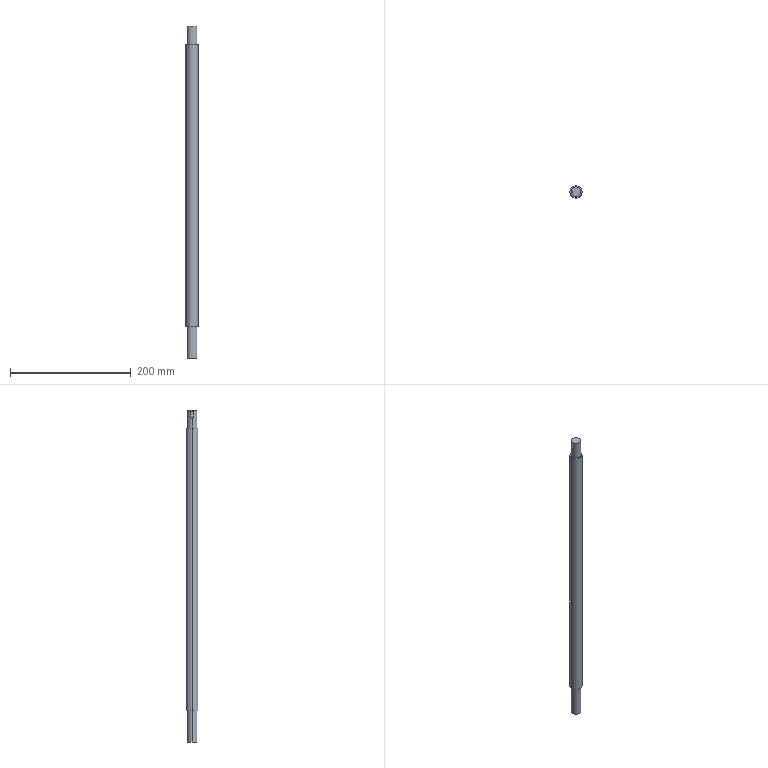Component | SolidWorks | LeadScrew-1 | 1 solid | 16 faces | box 20 x 20 x 550.64 mm | volume 163626 mm3 | cylinder 9 | plane 7 | commonest cylinder face diameters 16 x4 4 x3 20 x2
build123d program:
from build123d import *

# Parameters (mm, degrees)
SKETCH1_R           = 10
BOSS_EXTRUDE1_DEPTH = 529
SKETCH2_R           = 10
SKETCH2_R_2         = 8
CUT_EXTRUDE1_DEPTH  = 30
CUT_EXTRUDE2_START  = -30
SKETCH3_R           = 10
SKETCH3_R_2         = 8
CUT_EXTRUDE2_DEPTH  = 30
MOVE_FACE1_BY       = 21.644
CUT_EXTRUDE3_DEPTH  = 3


with BuildPart() as part:
    # Sketch1 → Boss-Extrude1 (new body)
    with BuildSketch(Plane.XY):
        with Locations((0, -208.707)):
            Circle(SKETCH1_R)
    extrude(amount=BOSS_EXTRUDE1_DEPTH)

    # Sketch2 → Cut-Extrude1 (cut)
    with BuildSketch(Plane(origin=(0, 0, 0), x_dir=(-1, 0, 0), z_dir=(0, 0, -1))):
        with Locations((0, -208.707)):
            Circle(SKETCH2_R)
        with Locations((0, -208.707)):
            Circle(SKETCH2_R_2, mode=Mode.SUBTRACT)
    extrude(amount=-CUT_EXTRUDE1_DEPTH, mode=Mode.SUBTRACT)

    # Sketch3 → Cut-Extrude2 (cut)
    with BuildSketch(Plane.XY.offset(529).offset(CUT_EXTRUDE2_START)):
        with Locations(Location((0, -208.707, 0), (0, 0, 180))):
            Circle(SKETCH3_R)
        with Locations(Location((0, -208.707, 0), (0, 0, 180))):
            Circle(SKETCH3_R_2, mode=Mode.SUBTRACT)
    extrude(amount=CUT_EXTRUDE2_DEPTH, mode=Mode.SUBTRACT)

    # Move Face1: a face moved outward by 21.644
    extrude(part.faces().sort_by_distance((0, -208.707, 529))[0], amount=MOVE_FACE1_BY, dir=(0, 0, 1))

    # Sketch4 → Cut-Extrude3 (cut)
    with BuildSketch(Plane(origin=(8, 0, 0), x_dir=(0, 0, -1), z_dir=(1, 0, 0))):
        with BuildLine():
            Line((-12, -206.707), (-4, -206.707))
            ThreePointArc((-4, -206.707), (-2, -208.707), (-4, -210.707))
            Line((-4, -210.707), (-12, -210.707))
            ThreePointArc((-12, -210.707), (-14, -208.707), (-12, -206.707))
        make_face()
    extrude(amount=-CUT_EXTRUDE3_DEPTH, mode=Mode.SUBTRACT)


solid = part.part

# Placed as in the assembly
solid = solid.moved(Location((0, 0, -102), (-180, 0, 180)))
STEP:
#1=CARTESIAN_POINT('',(-0.1969,-8.217,-4.094));
#2=VERTEX_POINT('',#1);
#3=CARTESIAN_POINT('',(-0.1969,-8.138,-4.173));
#4=VERTEX_POINT('',#3);
#5=CARTESIAN_POINT('',(-0.1969,-8.217,-4.173));
#6=DIRECTION('',(-1.,0.,0.));
#7=DIRECTION('',(0.,0.,1.));
#8=AXIS2_PLACEMENT_3D('',#5,#6,#7);
#9=CIRCLE('',#8,0.07874);
#10=EDGE_CURVE('',#2,#4,#9,.T.);
#11=ORIENTED_EDGE('',*,*,#10,.F.);
#12=CARTESIAN_POINT('',(-0.315,-8.217,-4.094));
#13=VERTEX_POINT('',#12);
#14=CARTESIAN_POINT('',(-0.1969,-8.217,-4.094));
#15=DIRECTION('',(-1.,0.,0.));
#16=VECTOR('',#15,39.37);
#17=LINE('',#14,#16);
#18=EDGE_CURVE('',#2,#13,#17,.T.);
#19=ORIENTED_EDGE('',*,*,#18,.T.);
#20=CARTESIAN_POINT('',(-0.305,-8.138,-4.173));
#21=VERTEX_POINT('',#20);
#22=CARTESIAN_POINT('',(-0.315,-8.217,-4.094));
#23=CARTESIAN_POINT('',(-0.315,-8.212,-4.094));
#24=CARTESIAN_POINT('',(-0.3148,-8.206,-4.095));
#25=CARTESIAN_POINT('',(-0.3143,-8.196,-4.097));
#26=CARTESIAN_POINT('',(-0.314,-8.191,-4.099));
#27=CARTESIAN_POINT('',(-0.3126,-8.177,-4.104));
#28=CARTESIAN_POINT('',(-0.3113,-8.168,-4.11));
#29=CARTESIAN_POINT('',(-0.3093,-8.158,-4.121));
#30=CARTESIAN_POINT('',(-0.3087,-8.154,-4.125));
#31=CARTESIAN_POINT('',(-0.3075,-8.149,-4.134));
#32=CARTESIAN_POINT('',(-0.3069,-8.146,-4.138));
#33=CARTESIAN_POINT('',(-0.306,-8.142,-4.148));
#34=CARTESIAN_POINT('',(-0.3056,-8.141,-4.153));
#35=CARTESIAN_POINT('',(-0.3051,-8.139,-4.163));
#36=CARTESIAN_POINT('',(-0.305,-8.138,-4.168));
#37=CARTESIAN_POINT('',(-0.305,-8.138,-4.173));
#38=B_SPLINE_CURVE_WITH_KNOTS('',3,(#22,#23,#24,#25,#26,#27,#28,#29,#30,#31,#32,#33,#34,#35,#36,#37),.UNSPECIFIED.,.F.,.F.,(4,2,2,2,2,2,2,4),(0.00314,0.003532,0.003924,0.004708,0.0051,0.005492,0.005884,0.006276),.UNSPECIFIED.);
#39=EDGE_CURVE('',#13,#21,#38,.T.);
#40=ORIENTED_EDGE('',*,*,#39,.T.);
#41=CARTESIAN_POINT('',(-0.1969,-8.138,-4.173));
#42=DIRECTION('',(-1.,0.,0.));
#43=VECTOR('',#42,39.37);
#44=LINE('',#41,#43);
#45=EDGE_CURVE('',#4,#21,#44,.T.);
#46=ORIENTED_EDGE('',*,*,#45,.F.);
#47=EDGE_LOOP('',(#11,#19,#40,#46));
#48=FACE_OUTER_BOUND('',#47,.T.);
#49=CARTESIAN_POINT('',(-0.1969,-8.217,-4.173));
#50=DIRECTION('',(-1.,0.,0.));
#51=DIRECTION('',(0.,0.,1.));
#52=AXIS2_PLACEMENT_3D('',#49,#50,#51);
#53=CYLINDRICAL_SURFACE('',#52,0.07874);
#54=ADVANCED_FACE('',(#48),#53,.F.);
#55=CARTESIAN_POINT('',(-0.315,-8.217,-23.661));
#56=VERTEX_POINT('',#55);
#57=CARTESIAN_POINT('',(0.315,-8.217,-23.661));
#58=VERTEX_POINT('',#57);
#59=CARTESIAN_POINT('',(0.,-8.217,-23.661));
#60=DIRECTION('',(0.,0.,-1.));
#61=DIRECTION('',(-1.,0.,0.));
#62=AXIS2_PLACEMENT_3D('',#59,#60,#61);
#63=CIRCLE('',#62,0.315);
#64=EDGE_CURVE('',#56,#58,#63,.T.);
#65=ORIENTED_EDGE('',*,*,#64,.T.);
#66=CARTESIAN_POINT('',(0.315,-8.217,-25.695));
#67=VERTEX_POINT('',#66);
#68=CARTESIAN_POINT('',(0.315,-8.217,-23.661));
#69=DIRECTION('',(0.,0.,-1.));
#70=VECTOR('',#69,39.37);
#71=LINE('',#68,#70);
#72=EDGE_CURVE('',#58,#67,#71,.T.);
#73=ORIENTED_EDGE('',*,*,#72,.T.);
#74=CARTESIAN_POINT('',(-0.315,-8.217,-25.695));
#75=VERTEX_POINT('',#74);
#76=CARTESIAN_POINT('',(0.,-8.217,-25.695));
#77=DIRECTION('',(0.,0.,-1.));
#78=DIRECTION('',(-1.,0.,0.));
#79=AXIS2_PLACEMENT_3D('',#76,#77,#78);
#80=CIRCLE('',#79,0.315);
#81=EDGE_CURVE('',#75,#67,#80,.T.);
#82=ORIENTED_EDGE('',*,*,#81,.F.);
#83=CARTESIAN_POINT('',(-0.315,-8.217,-23.661));
#84=DIRECTION('',(0.,0.,-1.));
#85=VECTOR('',#84,39.37);
#86=LINE('',#83,#85);
#87=EDGE_CURVE('',#56,#75,#86,.T.);
#88=ORIENTED_EDGE('',*,*,#87,.F.);
#89=EDGE_LOOP('',(#65,#73,#82,#88));
#90=FACE_OUTER_BOUND('',#89,.T.);
#91=CARTESIAN_POINT('',(0.,-8.217,-23.661));
#92=DIRECTION('',(0.,0.,-1.));
#93=DIRECTION('',(-1.,0.,0.));
#94=AXIS2_PLACEMENT_3D('',#91,#92,#93);
#95=CYLINDRICAL_SURFACE('',#94,0.315);
#96=ADVANCED_FACE('',(#90),#95,.T.);
#97=CARTESIAN_POINT('',(0.315,-8.217,-5.197));
#98=VERTEX_POINT('',#97);
#99=CARTESIAN_POINT('',(-0.315,-8.217,-5.197));
#100=VERTEX_POINT('',#99);
#101=CARTESIAN_POINT('',(0.,-8.217,-5.197));
#102=DIRECTION('',(0.,0.,1.));
#103=DIRECTION('',(1.,0.,0.));
#104=AXIS2_PLACEMENT_3D('',#101,#102,#103);
#105=CIRCLE('',#104,0.315);
#106=EDGE_CURVE('',#98,#100,#105,.T.);
#107=ORIENTED_EDGE('',*,*,#106,.T.);
#108=CARTESIAN_POINT('',(-0.315,-8.217,-4.567));
#109=VERTEX_POINT('',#108);
#110=CARTESIAN_POINT('',(-0.315,-8.217,-5.197));
#111=DIRECTION('',(0.,0.,1.));
#112=VECTOR('',#111,39.37);
#113=LINE('',#110,#112);
#114=EDGE_CURVE('',#100,#109,#113,.T.);
#115=ORIENTED_EDGE('',*,*,#114,.T.);
#116=CARTESIAN_POINT('',(-0.305,-8.138,-4.488));
#117=VERTEX_POINT('',#116);
#118=CARTESIAN_POINT('',(-0.305,-8.138,-4.488));
#119=CARTESIAN_POINT('',(-0.305,-8.138,-4.493));
#120=CARTESIAN_POINT('',(-0.3051,-8.139,-4.499));
#121=CARTESIAN_POINT('',(-0.3056,-8.141,-4.509));
#122=CARTESIAN_POINT('',(-0.306,-8.142,-4.514));
#123=CARTESIAN_POINT('',(-0.3069,-8.146,-4.523));
#124=CARTESIAN_POINT('',(-0.3075,-8.149,-4.528));
#125=CARTESIAN_POINT('',(-0.3087,-8.154,-4.536));
#126=CARTESIAN_POINT('',(-0.3094,-8.158,-4.54));
#127=CARTESIAN_POINT('',(-0.3113,-8.168,-4.551));
#128=CARTESIAN_POINT('',(-0.3126,-8.177,-4.557));
#129=CARTESIAN_POINT('',(-0.314,-8.191,-4.563));
#130=CARTESIAN_POINT('',(-0.3143,-8.196,-4.564));
#131=CARTESIAN_POINT('',(-0.3148,-8.207,-4.566));
#132=CARTESIAN_POINT('',(-0.315,-8.212,-4.567));
#133=CARTESIAN_POINT('',(-0.315,-8.217,-4.567));
#134=B_SPLINE_CURVE_WITH_KNOTS('',3,(#118,#119,#120,#121,#122,#123,#124,#125,#126,#127,#128,#129,#130,#131,#132,#133),.UNSPECIFIED.,.F.,.F.,(4,2,2,2,2,2,2,4),(0.,0.0003925,0.0007849,0.001177,0.00157,0.002355,0.002747,0.00314),.UNSPECIFIED.);
#135=EDGE_CURVE('',#117,#109,#134,.T.);
#136=ORIENTED_EDGE('',*,*,#135,.F.);
#137=CARTESIAN_POINT('',(-0.305,-8.138,-5.197));
#138=DIRECTION('',(0.,0.,-1.));
#139=VECTOR('',#138,39.37);
#140=LINE('',#137,#139);
#141=EDGE_CURVE('',#21,#117,#140,.T.);
#142=ORIENTED_EDGE('',*,*,#141,.F.);
#143=ORIENTED_EDGE('',*,*,#39,.F.);
#144=CARTESIAN_POINT('',(-0.315,-8.217,-4.016));
#145=VERTEX_POINT('',#144);
#146=CARTESIAN_POINT('',(-0.315,-8.217,-5.197));
#147=DIRECTION('',(0.,0.,1.));
#148=VECTOR('',#147,39.37);
#149=LINE('',#146,#148);
#150=EDGE_CURVE('',#13,#145,#149,.T.);
#151=ORIENTED_EDGE('',*,*,#150,.T.);
#152=CARTESIAN_POINT('',(0.315,-8.217,-4.016));
#153=VERTEX_POINT('',#152);
#154=CARTESIAN_POINT('',(0.,-8.217,-4.016));
#155=DIRECTION('',(0.,0.,1.));
#156=DIRECTION('',(1.,0.,0.));
#157=AXIS2_PLACEMENT_3D('',#154,#155,#156);
#158=CIRCLE('',#157,0.315);
#159=EDGE_CURVE('',#153,#145,#158,.T.);
#160=ORIENTED_EDGE('',*,*,#159,.F.);
#161=CARTESIAN_POINT('',(0.315,-8.217,-5.197));
#162=DIRECTION('',(0.,0.,1.));
#163=VECTOR('',#162,39.37);
#164=LINE('',#161,#163);
#165=EDGE_CURVE('',#98,#153,#164,.T.);
#166=ORIENTED_EDGE('',*,*,#165,.F.);
#167=EDGE_LOOP('',(#107,#115,#136,#142,#143,#151,#160,#166));
#168=FACE_OUTER_BOUND('',#167,.T.);
#169=CARTESIAN_POINT('',(0.,-8.217,-5.197));
#170=DIRECTION('',(0.,0.,1.));
#171=DIRECTION('',(1.,0.,0.));
#172=AXIS2_PLACEMENT_3D('',#169,#170,#171);
#173=CYLINDRICAL_SURFACE('',#172,0.315);
#174=ADVANCED_FACE('',(#168),#173,.T.);
#175=CARTESIAN_POINT('',(-0.3937,-8.217,-23.661));
#176=VERTEX_POINT('',#175);
#177=CARTESIAN_POINT('',(0.3937,-8.217,-23.661));
#178=VERTEX_POINT('',#177);
#179=CARTESIAN_POINT('',(0.,-8.217,-23.661));
#180=DIRECTION('',(0.,0.,-1.));
#181=DIRECTION('',(-1.,0.,0.));
#182=AXIS2_PLACEMENT_3D('',#179,#180,#181);
#183=CIRCLE('',#182,0.3937);
#184=EDGE_CURVE('',#176,#178,#183,.T.);
#185=ORIENTED_EDGE('',*,*,#184,.F.);
#186=CARTESIAN_POINT('',(-0.3937,-8.217,-5.197));
#187=VERTEX_POINT('',#186);
#188=CARTESIAN_POINT('',(-0.3937,-8.217,-24.843));
#189=DIRECTION('',(0.,0.,1.));
#190=VECTOR('',#189,39.37);
#191=LINE('',#188,#190);
#192=EDGE_CURVE('',#176,#187,#191,.T.);
#193=ORIENTED_EDGE('',*,*,#192,.T.);
#194=CARTESIAN_POINT('',(0.3937,-8.217,-5.197));
#195=VERTEX_POINT('',#194);
#196=CARTESIAN_POINT('',(0.,-8.217,-5.197));
#197=DIRECTION('',(0.,0.,1.));
#198=DIRECTION('',(1.,0.,0.));
#199=AXIS2_PLACEMENT_3D('',#196,#197,#198);
#200=CIRCLE('',#199,0.3937);
#201=EDGE_CURVE('',#195,#187,#200,.T.);
#202=ORIENTED_EDGE('',*,*,#201,.F.);
#203=CARTESIAN_POINT('',(0.3937,-8.217,-24.843));
#204=DIRECTION('',(0.,0.,1.));
#205=VECTOR('',#204,39.37);
#206=LINE('',#203,#205);
#207=EDGE_CURVE('',#178,#195,#206,.T.);
#208=ORIENTED_EDGE('',*,*,#207,.F.);
#209=EDGE_LOOP('',(#185,#193,#202,#208));
#210=FACE_OUTER_BOUND('',#209,.T.);
#211=CARTESIAN_POINT('',(0.,-8.217,-24.843));
#212=DIRECTION('',(0.,0.,1.));
#213=DIRECTION('',(1.,0.,0.));
#214=AXIS2_PLACEMENT_3D('',#211,#212,#213);
#215=CYLINDRICAL_SURFACE('',#214,0.3937);
#216=ADVANCED_FACE('',(#210),#215,.T.);
#217=ORIENTED_EDGE('',*,*,#192,.F.);
#218=CARTESIAN_POINT('',(0.,-8.217,-23.661));
#219=DIRECTION('',(0.,0.,-1.));
#220=DIRECTION('',(-1.,0.,0.));
#221=AXIS2_PLACEMENT_3D('',#218,#219,#220);
#222=CIRCLE('',#221,0.3937);
#223=EDGE_CURVE('',#178,#176,#222,.T.);
#224=ORIENTED_EDGE('',*,*,#223,.F.);
#225=ORIENTED_EDGE('',*,*,#207,.T.);
#226=CARTESIAN_POINT('',(0.,-8.217,-5.197));
#227=DIRECTION('',(0.,0.,1.));
#228=DIRECTION('',(1.,0.,0.));
#229=AXIS2_PLACEMENT_3D('',#226,#227,#228);
#230=CIRCLE('',#229,0.3937);
#231=EDGE_CURVE('',#187,#195,#230,.T.);
#232=ORIENTED_EDGE('',*,*,#231,.F.);
#233=EDGE_LOOP('',(#217,#224,#225,#232));
#234=FACE_OUTER_BOUND('',#233,.T.);
#235=CARTESIAN_POINT('',(0.,-8.217,-24.843));
#236=DIRECTION('',(0.,0.,1.));
#237=DIRECTION('',(1.,0.,0.));
#238=AXIS2_PLACEMENT_3D('',#235,#236,#237);
#239=CYLINDRICAL_SURFACE('',#238,0.3937);
#240=ADVANCED_FACE('',(#234),#239,.T.);
#241=ORIENTED_EDGE('',*,*,#106,.F.);
#242=CARTESIAN_POINT('',(0.,-8.217,-5.197));
#243=DIRECTION('',(0.,0.,1.));
#244=DIRECTION('',(1.,0.,0.));
#245=AXIS2_PLACEMENT_3D('',#242,#243,#244);
#246=CIRCLE('',#245,0.315);
#247=EDGE_CURVE('',#100,#98,#246,.T.);
#248=ORIENTED_EDGE('',*,*,#247,.F.);
#249=EDGE_LOOP('',(#241,#248));
#250=FACE_BOUND('',#249,.T.);
#251=ORIENTED_EDGE('',*,*,#201,.T.);
#252=ORIENTED_EDGE('',*,*,#231,.T.);
#253=EDGE_LOOP('',(#251,#252));
#254=FACE_OUTER_BOUND('',#253,.T.);
#255=CARTESIAN_POINT('',(0.,-8.217,-5.197));
#256=DIRECTION('',(0.,0.,1.));
#257=DIRECTION('',(1.,0.,0.));
#258=AXIS2_PLACEMENT_3D('',#255,#256,#257);
#259=PLANE('',#258);
#260=ADVANCED_FACE('',(#250,#254),#259,.T.);
#261=ORIENTED_EDGE('',*,*,#114,.F.);
#262=ORIENTED_EDGE('',*,*,#247,.T.);
#263=ORIENTED_EDGE('',*,*,#165,.T.);
#264=CARTESIAN_POINT('',(0.,-8.217,-4.016));
#265=DIRECTION('',(0.,0.,1.));
#266=DIRECTION('',(1.,0.,0.));
#267=AXIS2_PLACEMENT_3D('',#264,#265,#266);
#268=CIRCLE('',#267,0.315);
#269=EDGE_CURVE('',#145,#153,#268,.T.);
#270=ORIENTED_EDGE('',*,*,#269,.F.);
#271=ORIENTED_EDGE('',*,*,#150,.F.);
#272=CARTESIAN_POINT('',(-0.305,-8.296,-4.173));
#273=VERTEX_POINT('',#272);
#274=CARTESIAN_POINT('',(-0.305,-8.296,-4.173));
#275=CARTESIAN_POINT('',(-0.305,-8.296,-4.168));
#276=CARTESIAN_POINT('',(-0.3051,-8.295,-4.163));
#277=CARTESIAN_POINT('',(-0.3056,-8.293,-4.153));
#278=CARTESIAN_POINT('',(-0.306,-8.292,-4.148));
#279=CARTESIAN_POINT('',(-0.3069,-8.288,-4.138));
#280=CARTESIAN_POINT('',(-0.3075,-8.285,-4.134));
#281=CARTESIAN_POINT('',(-0.3087,-8.279,-4.125));
#282=CARTESIAN_POINT('',(-0.3094,-8.276,-4.121));
#283=CARTESIAN_POINT('',(-0.3113,-8.265,-4.11));
#284=CARTESIAN_POINT('',(-0.3126,-8.256,-4.104));
#285=CARTESIAN_POINT('',(-0.314,-8.242,-4.099));
#286=CARTESIAN_POINT('',(-0.3143,-8.237,-4.097));
#287=CARTESIAN_POINT('',(-0.3148,-8.227,-4.095));
#288=CARTESIAN_POINT('',(-0.315,-8.222,-4.094));
#289=CARTESIAN_POINT('',(-0.315,-8.217,-4.094));
#290=B_SPLINE_CURVE_WITH_KNOTS('',3,(#274,#275,#276,#277,#278,#279,#280,#281,#282,#283,#284,#285,#286,#287,#288,#289),.UNSPECIFIED.,.F.,.F.,(4,2,2,2,2,2,2,4),(0.,0.0003925,0.0007849,0.001177,0.00157,0.002355,0.002747,0.00314),.UNSPECIFIED.);
#291=EDGE_CURVE('',#273,#13,#290,.T.);
#292=ORIENTED_EDGE('',*,*,#291,.F.);
#293=CARTESIAN_POINT('',(-0.305,-8.296,-4.488));
#294=VERTEX_POINT('',#293);
#295=CARTESIAN_POINT('',(-0.305,-8.296,-5.197));
#296=DIRECTION('',(0.,0.,1.));
#297=VECTOR('',#296,39.37);
#298=LINE('',#295,#297);
#299=EDGE_CURVE('',#294,#273,#298,.T.);
#300=ORIENTED_EDGE('',*,*,#299,.F.);
#301=CARTESIAN_POINT('',(-0.315,-8.217,-4.567));
#302=CARTESIAN_POINT('',(-0.315,-8.222,-4.567));
#303=CARTESIAN_POINT('',(-0.3148,-8.227,-4.566));
#304=CARTESIAN_POINT('',(-0.3143,-8.237,-4.564));
#305=CARTESIAN_POINT('',(-0.314,-8.242,-4.563));
#306=CARTESIAN_POINT('',(-0.3126,-8.257,-4.557));
#307=CARTESIAN_POINT('',(-0.3113,-8.265,-4.551));
#308=CARTESIAN_POINT('',(-0.3093,-8.276,-4.54));
#309=CARTESIAN_POINT('',(-0.3087,-8.279,-4.536));
#310=CARTESIAN_POINT('',(-0.3075,-8.285,-4.528));
#311=CARTESIAN_POINT('',(-0.3069,-8.288,-4.523));
#312=CARTESIAN_POINT('',(-0.306,-8.292,-4.514));
#313=CARTESIAN_POINT('',(-0.3056,-8.293,-4.509));
#314=CARTESIAN_POINT('',(-0.3051,-8.295,-4.499));
#315=CARTESIAN_POINT('',(-0.305,-8.296,-4.493));
#316=CARTESIAN_POINT('',(-0.305,-8.296,-4.488));
#317=B_SPLINE_CURVE_WITH_KNOTS('',3,(#301,#302,#303,#304,#305,#306,#307,#308,#309,#310,#311,#312,#313,#314,#315,#316),.UNSPECIFIED.,.F.,.F.,(4,2,2,2,2,2,2,4),(0.00314,0.003532,0.003924,0.004708,0.0051,0.005492,0.005884,0.006276),.UNSPECIFIED.);
#318=EDGE_CURVE('',#109,#294,#317,.T.);
#319=ORIENTED_EDGE('',*,*,#318,.F.);
#320=EDGE_LOOP('',(#261,#262,#263,#270,#271,#292,#300,#319));
#321=FACE_OUTER_BOUND('',#320,.T.);
#322=CARTESIAN_POINT('',(0.,-8.217,-5.197));
#323=DIRECTION('',(0.,0.,1.));
#324=DIRECTION('',(1.,0.,0.));
#325=AXIS2_PLACEMENT_3D('',#322,#323,#324);
#326=CYLINDRICAL_SURFACE('',#325,0.315);
#327=ADVANCED_FACE('',(#321),#326,.T.);
#328=ORIENTED_EDGE('',*,*,#159,.T.);
#329=ORIENTED_EDGE('',*,*,#269,.T.);
#330=EDGE_LOOP('',(#328,#329));
#331=FACE_OUTER_BOUND('',#330,.T.);
#332=CARTESIAN_POINT('',(0.,-8.217,-4.016));
#333=DIRECTION('',(0.,0.,-1.));
#334=DIRECTION('',(-1.,0.,0.));
#335=AXIS2_PLACEMENT_3D('',#332,#333,#334);
#336=PLANE('',#335);
#337=ADVANCED_FACE('',(#331),#336,.F.);
#338=ORIENTED_EDGE('',*,*,#72,.F.);
#339=CARTESIAN_POINT('',(0.,-8.217,-23.661));
#340=DIRECTION('',(0.,0.,-1.));
#341=DIRECTION('',(-1.,0.,0.));
#342=AXIS2_PLACEMENT_3D('',#339,#340,#341);
#343=CIRCLE('',#342,0.315);
#344=EDGE_CURVE('',#58,#56,#343,.T.);
#345=ORIENTED_EDGE('',*,*,#344,.T.);
#346=ORIENTED_EDGE('',*,*,#87,.T.);
#347=CARTESIAN_POINT('',(0.,-8.217,-25.695));
#348=DIRECTION('',(0.,0.,-1.));
#349=DIRECTION('',(-1.,0.,0.));
#350=AXIS2_PLACEMENT_3D('',#347,#348,#349);
#351=CIRCLE('',#350,0.315);
#352=EDGE_CURVE('',#67,#75,#351,.T.);
#353=ORIENTED_EDGE('',*,*,#352,.F.);
#354=EDGE_LOOP('',(#338,#345,#346,#353));
#355=FACE_OUTER_BOUND('',#354,.T.);
#356=CARTESIAN_POINT('',(0.,-8.217,-23.661));
#357=DIRECTION('',(0.,0.,-1.));
#358=DIRECTION('',(-1.,0.,0.));
#359=AXIS2_PLACEMENT_3D('',#356,#357,#358);
#360=CYLINDRICAL_SURFACE('',#359,0.315);
#361=ADVANCED_FACE('',(#355),#360,.T.);
#362=ORIENTED_EDGE('',*,*,#64,.F.);
#363=ORIENTED_EDGE('',*,*,#344,.F.);
#364=EDGE_LOOP('',(#362,#363));
#365=FACE_BOUND('',#364,.T.);
#366=ORIENTED_EDGE('',*,*,#223,.T.);
#367=ORIENTED_EDGE('',*,*,#184,.T.);
#368=EDGE_LOOP('',(#366,#367));
#369=FACE_OUTER_BOUND('',#368,.T.);
#370=CARTESIAN_POINT('',(0.,0.,-23.661));
#371=DIRECTION('',(0.,0.,-1.));
#372=DIRECTION('',(-1.,0.,0.));
#373=AXIS2_PLACEMENT_3D('',#370,#371,#372);
#374=PLANE('',#373);
#375=ADVANCED_FACE('',(#365,#369),#374,.T.);
#376=ORIENTED_EDGE('',*,*,#81,.T.);
#377=ORIENTED_EDGE('',*,*,#352,.T.);
#378=EDGE_LOOP('',(#376,#377));
#379=FACE_OUTER_BOUND('',#378,.T.);
#380=CARTESIAN_POINT('',(0.,-8.217,-25.695));
#381=DIRECTION('',(0.,0.,-1.));
#382=DIRECTION('',(-1.,0.,0.));
#383=AXIS2_PLACEMENT_3D('',#380,#381,#382);
#384=PLANE('',#383);
#385=ADVANCED_FACE('',(#379),#384,.T.);
#386=CARTESIAN_POINT('',(-0.1969,-8.138,-4.488));
#387=VERTEX_POINT('',#386);
#388=CARTESIAN_POINT('',(-0.1969,-8.138,-4.488));
#389=DIRECTION('',(-1.,0.,0.));
#390=VECTOR('',#389,39.37);
#391=LINE('',#388,#390);
#392=EDGE_CURVE('',#387,#117,#391,.T.);
#393=ORIENTED_EDGE('',*,*,#392,.T.);
#394=ORIENTED_EDGE('',*,*,#135,.T.);
#395=ORIENTED_EDGE('',*,*,#318,.T.);
#396=CARTESIAN_POINT('',(-0.1969,-8.296,-4.488));
#397=VERTEX_POINT('',#396);
#398=CARTESIAN_POINT('',(-0.1969,-8.296,-4.488));
#399=DIRECTION('',(-1.,0.,0.));
#400=VECTOR('',#399,39.37);
#401=LINE('',#398,#400);
#402=EDGE_CURVE('',#397,#294,#401,.T.);
#403=ORIENTED_EDGE('',*,*,#402,.F.);
#404=CARTESIAN_POINT('',(-0.1969,-8.217,-4.488));
#405=DIRECTION('',(-1.,0.,0.));
#406=DIRECTION('',(0.,0.,1.));
#407=AXIS2_PLACEMENT_3D('',#404,#405,#406);
#408=CIRCLE('',#407,0.07874);
#409=EDGE_CURVE('',#387,#397,#408,.T.);
#410=ORIENTED_EDGE('',*,*,#409,.F.);
#411=EDGE_LOOP('',(#393,#394,#395,#403,#410));
#412=FACE_OUTER_BOUND('',#411,.T.);
#413=CARTESIAN_POINT('',(-0.1969,-8.217,-4.488));
#414=DIRECTION('',(-1.,0.,0.));
#415=DIRECTION('',(0.,0.,1.));
#416=AXIS2_PLACEMENT_3D('',#413,#414,#415);
#417=CYLINDRICAL_SURFACE('',#416,0.07874);
#418=ADVANCED_FACE('',(#412),#417,.F.);
#419=ORIENTED_EDGE('',*,*,#141,.T.);
#420=ORIENTED_EDGE('',*,*,#392,.F.);
#421=CARTESIAN_POINT('',(-0.1969,-8.138,-4.488));
#422=DIRECTION('',(0.,0.,-1.));
#423=VECTOR('',#422,39.37);
#424=LINE('',#421,#423);
#425=EDGE_CURVE('',#4,#387,#424,.T.);
#426=ORIENTED_EDGE('',*,*,#425,.F.);
#427=ORIENTED_EDGE('',*,*,#45,.T.);
#428=EDGE_LOOP('',(#419,#420,#426,#427));
#429=FACE_OUTER_BOUND('',#428,.T.);
#430=CARTESIAN_POINT('',(-0.1969,-8.138,-4.488));
#431=DIRECTION('',(0.,1.,0.));
#432=DIRECTION('',(0.,0.,-1.));
#433=AXIS2_PLACEMENT_3D('',#430,#431,#432);
#434=PLANE('',#433);
#435=ADVANCED_FACE('',(#429),#434,.F.);
#436=ORIENTED_EDGE('',*,*,#18,.F.);
#437=CARTESIAN_POINT('',(-0.1969,-8.296,-4.173));
#438=VERTEX_POINT('',#437);
#439=CARTESIAN_POINT('',(-0.1969,-8.217,-4.173));
#440=DIRECTION('',(-1.,0.,0.));
#441=DIRECTION('',(0.,0.,1.));
#442=AXIS2_PLACEMENT_3D('',#439,#440,#441);
#443=CIRCLE('',#442,0.07874);
#444=EDGE_CURVE('',#438,#2,#443,.T.);
#445=ORIENTED_EDGE('',*,*,#444,.F.);
#446=CARTESIAN_POINT('',(-0.1969,-8.296,-4.173));
#447=DIRECTION('',(-1.,0.,0.));
#448=VECTOR('',#447,39.37);
#449=LINE('',#446,#448);
#450=EDGE_CURVE('',#438,#273,#449,.T.);
#451=ORIENTED_EDGE('',*,*,#450,.T.);
#452=ORIENTED_EDGE('',*,*,#291,.T.);
#453=EDGE_LOOP('',(#436,#445,#451,#452));
#454=FACE_OUTER_BOUND('',#453,.T.);
#455=CARTESIAN_POINT('',(-0.1969,-8.217,-4.173));
#456=DIRECTION('',(-1.,0.,0.));
#457=DIRECTION('',(0.,0.,1.));
#458=AXIS2_PLACEMENT_3D('',#455,#456,#457);
#459=CYLINDRICAL_SURFACE('',#458,0.07874);
#460=ADVANCED_FACE('',(#454),#459,.F.);
#461=ORIENTED_EDGE('',*,*,#299,.T.);
#462=ORIENTED_EDGE('',*,*,#450,.F.);
#463=CARTESIAN_POINT('',(-0.1969,-8.296,-4.488));
#464=DIRECTION('',(0.,0.,1.));
#465=VECTOR('',#464,39.37);
#466=LINE('',#463,#465);
#467=EDGE_CURVE('',#397,#438,#466,.T.);
#468=ORIENTED_EDGE('',*,*,#467,.F.);
#469=ORIENTED_EDGE('',*,*,#402,.T.);
#470=EDGE_LOOP('',(#461,#462,#468,#469));
#471=FACE_OUTER_BOUND('',#470,.T.);
#472=CARTESIAN_POINT('',(-0.1969,-8.296,-4.488));
#473=DIRECTION('',(0.,-1.,0.));
#474=DIRECTION('',(0.,0.,1.));
#475=AXIS2_PLACEMENT_3D('',#472,#473,#474);
#476=PLANE('',#475);
#477=ADVANCED_FACE('',(#471),#476,.F.);
#478=ORIENTED_EDGE('',*,*,#409,.T.);
#479=ORIENTED_EDGE('',*,*,#467,.T.);
#480=ORIENTED_EDGE('',*,*,#444,.T.);
#481=ORIENTED_EDGE('',*,*,#10,.T.);
#482=ORIENTED_EDGE('',*,*,#425,.T.);
#483=EDGE_LOOP('',(#478,#479,#480,#481,#482));
#484=FACE_OUTER_BOUND('',#483,.T.);
#485=CARTESIAN_POINT('',(-0.1969,-8.217,-4.488));
#486=DIRECTION('',(-1.,0.,0.));
#487=DIRECTION('',(0.,0.,1.));
#488=AXIS2_PLACEMENT_3D('',#485,#486,#487);
#489=PLANE('',#488);
#490=ADVANCED_FACE('',(#484),#489,.T.);
#491=CLOSED_SHELL('',(#54,#96,#174,#216,#240,#260,#327,#337,#361,#375,#385,#418,#435,#460,#477,#490));
#492=MANIFOLD_SOLID_BREP('',#491);
#493=CARTESIAN_POINT('',(0.,0.,0.));
#494=DIRECTION('',(0.,0.,1.));
#495=DIRECTION('',(1.,0.,0.));
#496=AXIS2_PLACEMENT_3D('',#493,#494,#495);
#497=(LENGTH_UNIT()NAMED_UNIT(*)SI_UNIT($,.METRE.));
#498=LENGTH_MEASURE_WITH_UNIT(LENGTH_MEASURE(0.0254),#497);
#499=DIMENSIONAL_EXPONENTS(1.,0.,0.,0.,0.,0.,0.);
#500=(CONVERSION_BASED_UNIT('',#498)LENGTH_UNIT()NAMED_UNIT(#499));
#501=UNCERTAINTY_MEASURE_WITH_UNIT(LENGTH_MEASURE(0.00001),#500,'','');
#502=(NAMED_UNIT(*)PLANE_ANGLE_UNIT()SI_UNIT($,.RADIAN.));
#503=(NAMED_UNIT(*)SI_UNIT($,.STERADIAN.)SOLID_ANGLE_UNIT());
#504=(GEOMETRIC_REPRESENTATION_CONTEXT(3)GLOBAL_UNCERTAINTY_ASSIGNED_CONTEXT((#501))GLOBAL_UNIT_ASSIGNED_CONTEXT((#500,#502,#503))REPRESENTATION_CONTEXT('',''));
#505=ADVANCED_BREP_SHAPE_REPRESENTATION('',(#492,#496),#504);
#506=COLOUR_RGB('',0.7922,0.8196,0.9333);
#507=FILL_AREA_STYLE_COLOUR('',#506);
#508=FILL_AREA_STYLE('',(#507));
#509=SURFACE_STYLE_FILL_AREA(#508);
#510=SURFACE_SIDE_STYLE('',(#509));
#511=SURFACE_STYLE_USAGE(.BOTH.,#510);
#512=PRESENTATION_STYLE_ASSIGNMENT((#511));
#513=STYLED_ITEM('',(#512),#492);
#514=PRESENTATION_LAYER_ASSIGNMENT('','',(#513));
#515=(LENGTH_UNIT()NAMED_UNIT(*)SI_UNIT($,.METRE.));
#516=LENGTH_MEASURE_WITH_UNIT(LENGTH_MEASURE(0.0254),#515);
#517=DIMENSIONAL_EXPONENTS(1.,0.,0.,0.,0.,0.,0.);
#518=(CONVERSION_BASED_UNIT('',#516)LENGTH_UNIT()NAMED_UNIT(#517));
#519=UNCERTAINTY_MEASURE_WITH_UNIT(LENGTH_MEASURE(0.00001),#518,'','');
#520=(NAMED_UNIT(*)PLANE_ANGLE_UNIT()SI_UNIT($,.RADIAN.));
#521=(NAMED_UNIT(*)SI_UNIT($,.STERADIAN.)SOLID_ANGLE_UNIT());
#522=(GEOMETRIC_REPRESENTATION_CONTEXT(3)GLOBAL_UNCERTAINTY_ASSIGNED_CONTEXT((#519))GLOBAL_UNIT_ASSIGNED_CONTEXT((#518,#520,#521))REPRESENTATION_CONTEXT('',''));
#523=MECHANICAL_DESIGN_GEOMETRIC_PRESENTATION_REPRESENTATION('',(#513),#522);